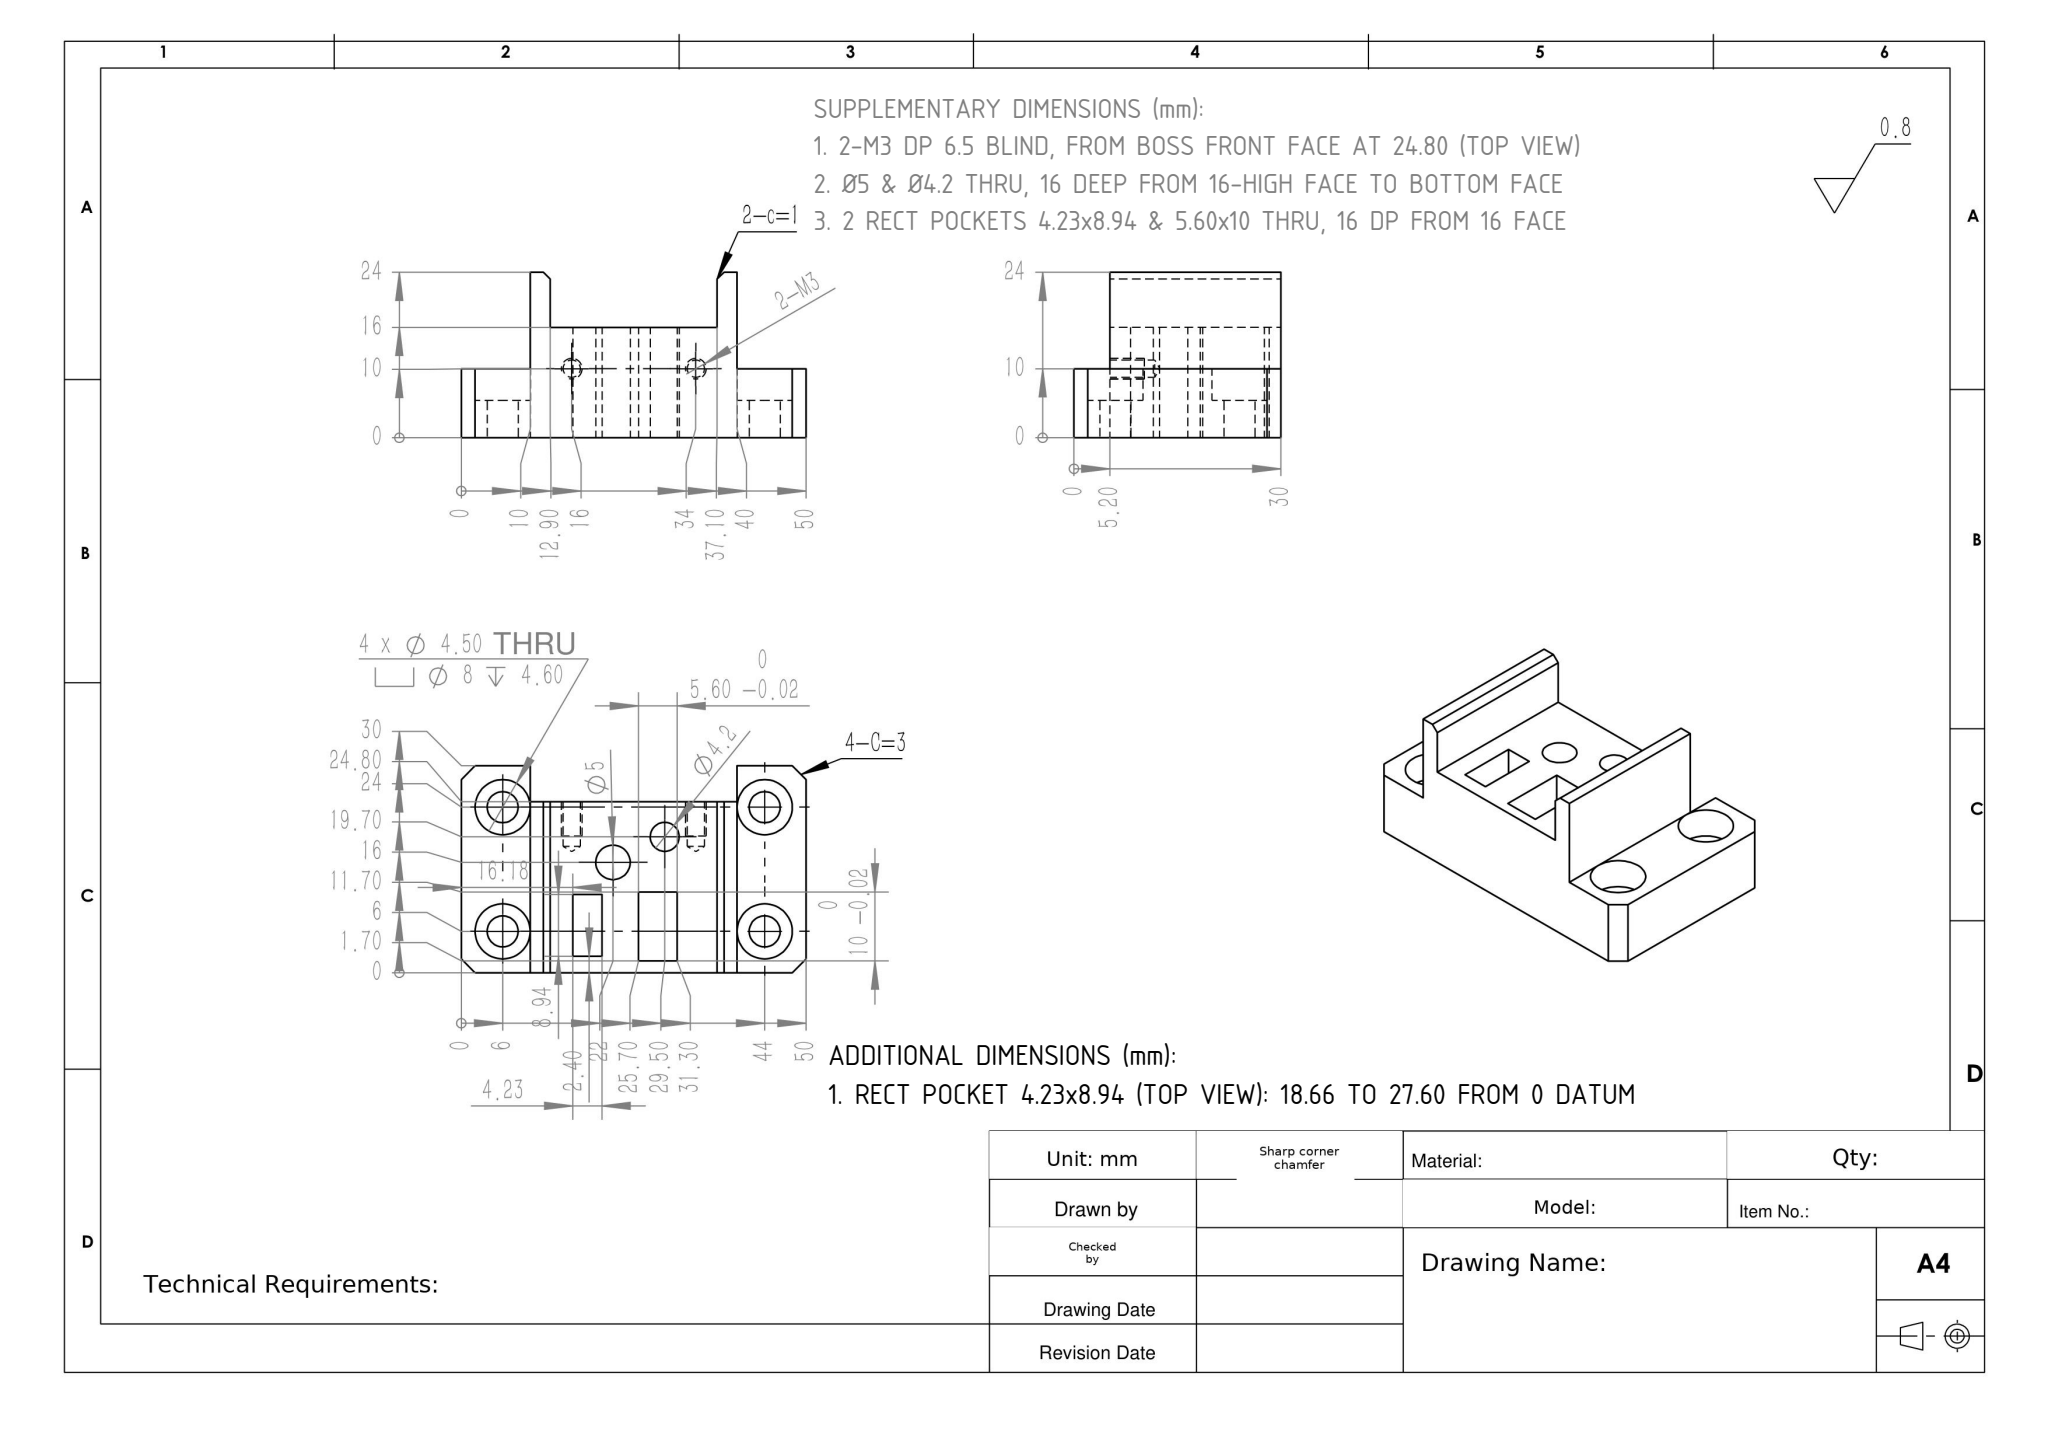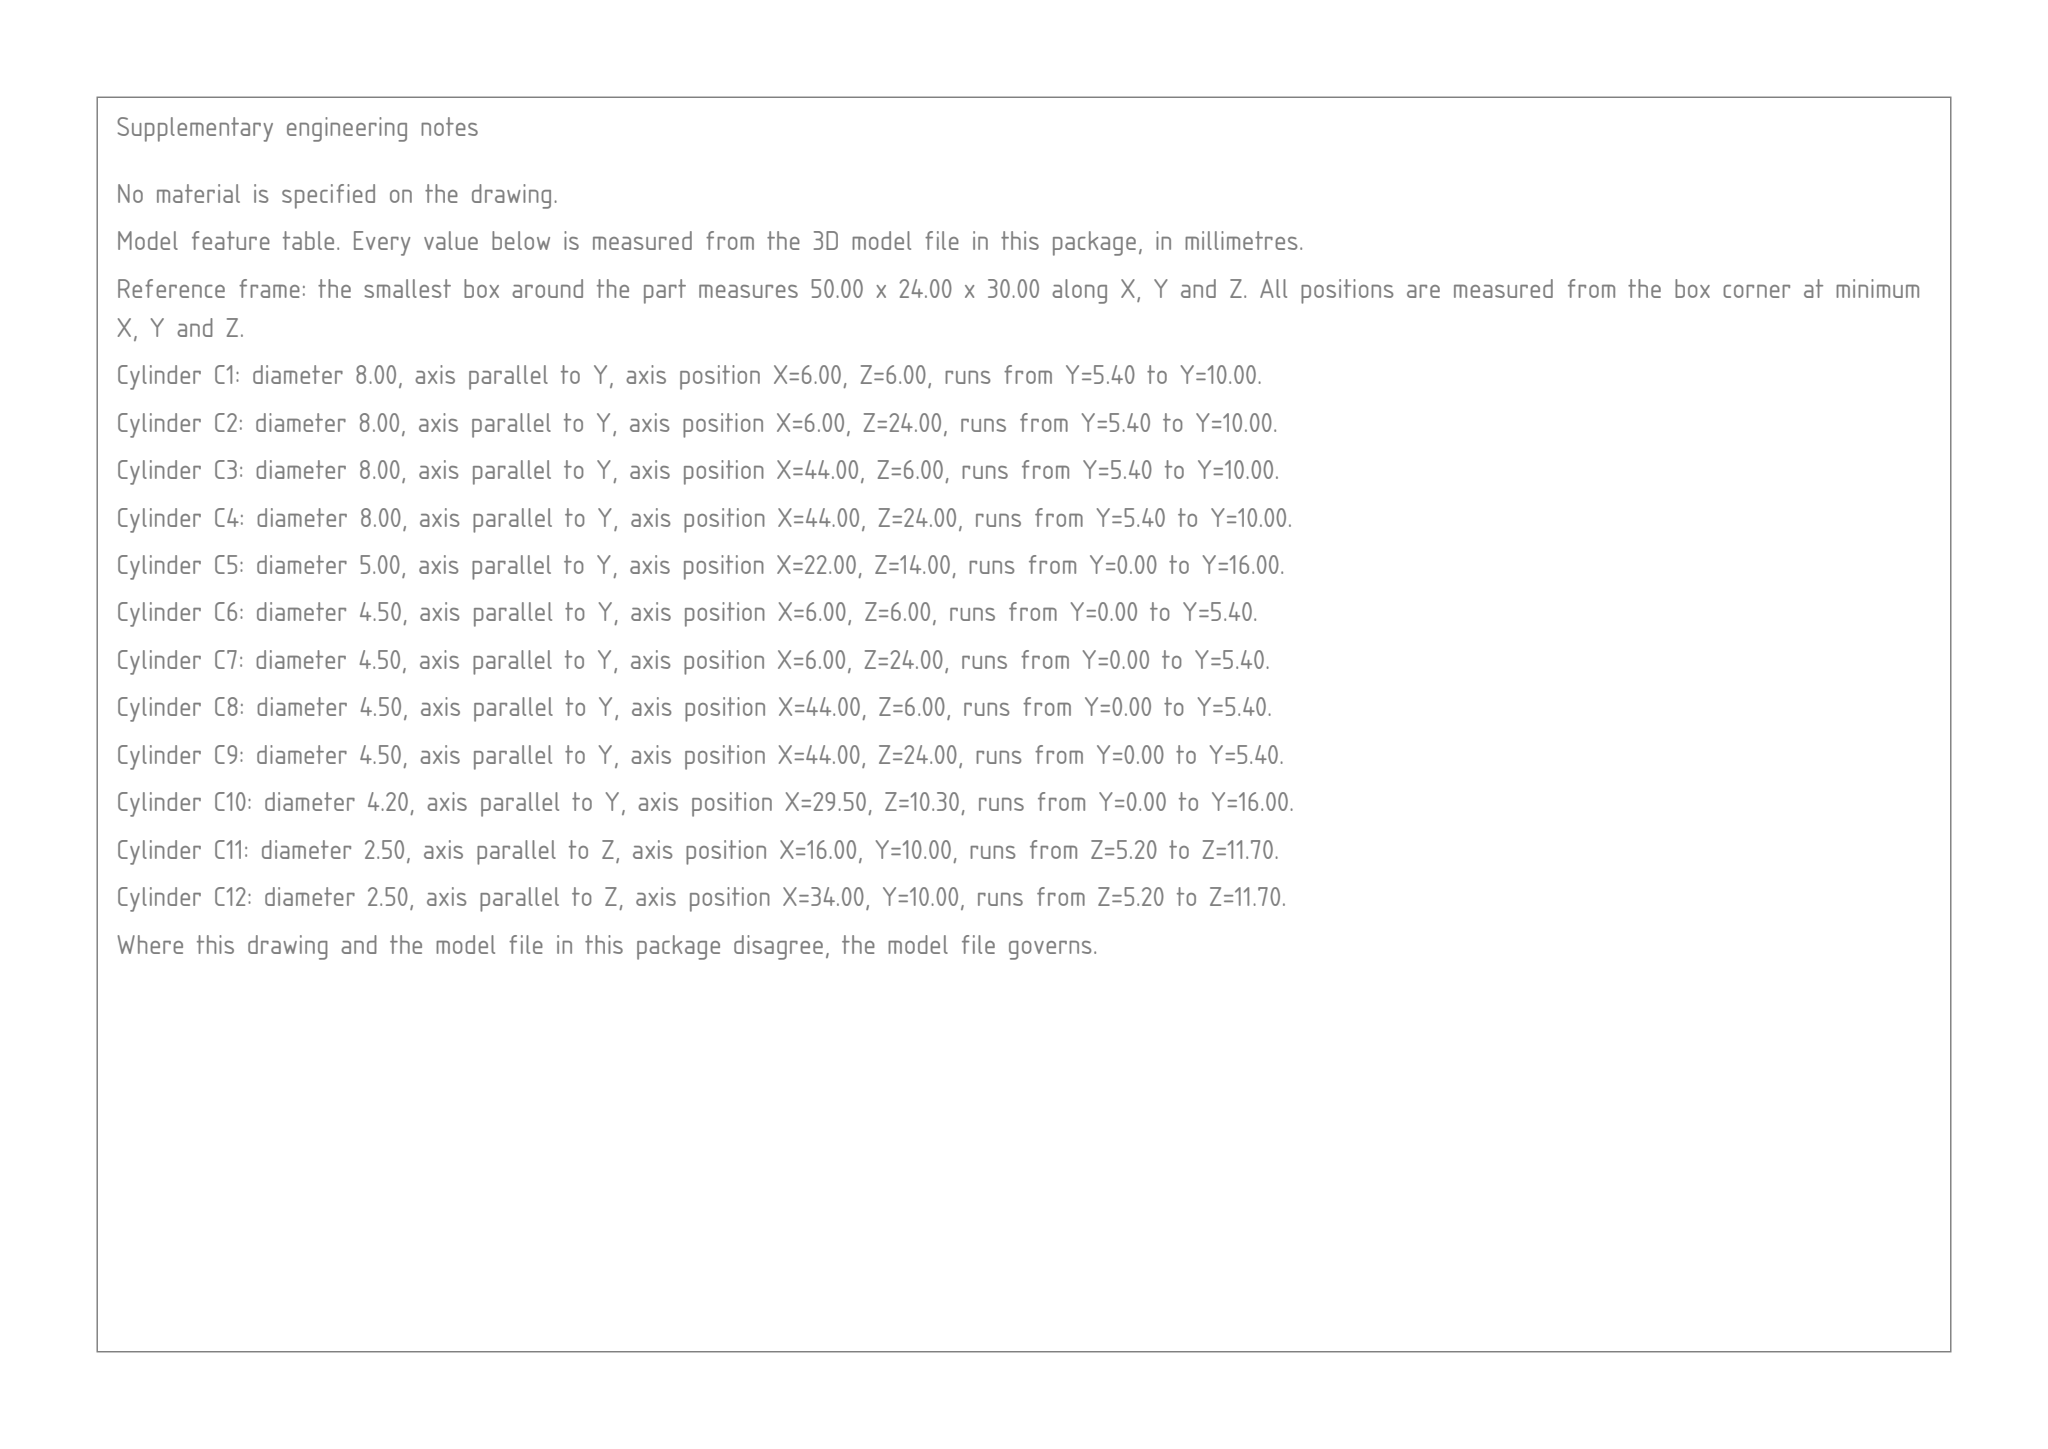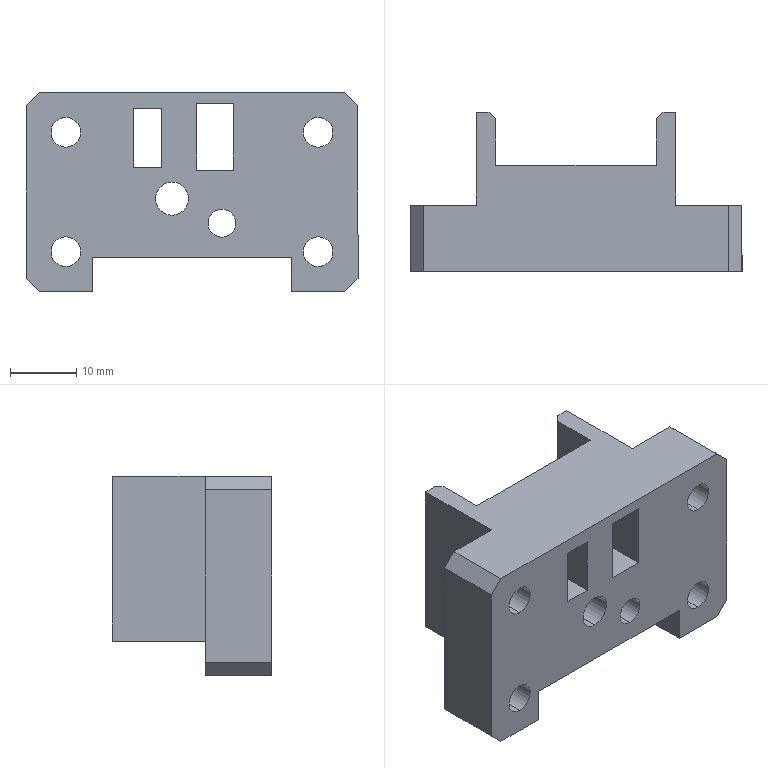Part | SolidWorks | mm | 1 solid | 64 faces | box 50 x 24 x 30 mm | volume 15578 mm3 | plane 36 | cylinder 24 | cone 4 | commonest cylinder face diameters 8 x8 4.5 x8 2.5 x4 5 x2 4.2 x2
build123d program:
from build123d import *

# Parameters (mm, degrees)
SKETCH1_W                                           = 50
SKETCH1_H                                           = 24
BOSS_EXTRUDE1_DEPTH                                 = 30
SKETCH2_W                                           = 10
SKETCH2_H                                           = 14
CUT_EXTRUDE1_DEPTH                                  = 64.056
SKETCH3_W                                           = 24.2
SKETCH3_H                                           = 8
CUT_EXTRUDE2_DEPTH                                  = 24.8
CHAMFER2_SIZE                                       = 2
SKETCH5_R                                           = 2.1
CUT_EXTRUDE3_DEPTH                                  = 64.056
HOLE_SIZE_TYPE_1_OF_SOCKET_HEAD_CAP_SCR_D           = 4.5
HOLE_SIZE_TYPE_1_OF_SOCKET_HEAD_CAP_SCR_CBORE_D     = 8
HOLE_SIZE_TYPE_1_OF_SOCKET_HEAD_CAP_SCR_CBORE_DEPTH = 4.6
CHAMFER3_SIZE                                       = 1
SKETCH12_W                                          = 5.6
SKETCH12_H                                          = 10
CUT_EXTRUDE5_DEPTH                                  = 61.465
SKETCH13_W                                          = 30
SKETCH13_H                                          = 5.2
CUT_EXTRUDE6_DEPTH                                  = 64.056
M3_TAPPED_HOLE1_D                                   = 2.5
M3_TAPPED_HOLE1_DEPTH                               = 6.5
M3_TAPPED_HOLE1_TIP                                 = 0.7511
CUT_EXTRUDE7_DEPTH                                  = 10
CUT_EXTRUDE7_DEPTH_BACK                             = 60.967
SKETCH16_R                                          = 2.5
SKETCH17_W                                          = 4.233
SKETCH17_H                                          = 8.941
CUT_EXTRUDE8_DEPTH                                  = 27


with BuildPart() as part:
    # Sketch1 → Boss-Extrude1 (new body)
    with BuildSketch(Plane.XY):
        with Locations((25, 12)):
            Rectangle(SKETCH1_W, SKETCH1_H)
    extrude(amount=BOSS_EXTRUDE1_DEPTH)

    # Sketch2 → Cut-Extrude1 (cut, through all)
    with BuildSketch(Plane.XY.offset(30)):
        with Locations((5, 17)):
            Rectangle(SKETCH2_W, SKETCH2_H)
        with Locations((45, 17)):
            Rectangle(SKETCH2_W, SKETCH2_H)
    extrude(amount=-CUT_EXTRUDE1_DEPTH, mode=Mode.SUBTRACT)

    # Sketch3 → Cut-Extrude2 (cut)
    with BuildSketch(Plane.XY.offset(30)):
        with Locations((25, 20)):
            Rectangle(SKETCH3_W, SKETCH3_H)
    extrude(amount=-CUT_EXTRUDE2_DEPTH, mode=Mode.SUBTRACT)

    # Chamfer2
    chamfer2_edges = [part.edges().sort_by_distance(p)[0] for p in [
        (50, 5, 30),
        (0, 5, 0),
        (0, 5, 30),
        (50, 5, 0),
    ]]
    chamfer(chamfer2_edges, length=CHAMFER2_SIZE)

    # Sketch5 → Cut-Extrude3 (cut, through all)
    with BuildSketch(Plane(origin=(0, 0, 0), x_dir=(-1, 0, 0), z_dir=(0, -1, 0))):
        with Locations(Location((-29.5, -10.3, 0), (0, 0, 90))):
            Circle(SKETCH5_R)
    extrude(amount=-CUT_EXTRUDE3_DEPTH, mode=Mode.SUBTRACT)

    # Hole Size _Type 1 of Socket Head Cap Scr (through all)
    with Locations(Plane(origin=(6, 10, 6), x_dir=(0, 0, 1), z_dir=(0, 1, 0))):
        with Locations((0, 0), (18, 0), (0, 38), (18, 38)):
            CounterBoreHole(HOLE_SIZE_TYPE_1_OF_SOCKET_HEAD_CAP_SCR_D / 2, HOLE_SIZE_TYPE_1_OF_SOCKET_HEAD_CAP_SCR_CBORE_D / 2, HOLE_SIZE_TYPE_1_OF_SOCKET_HEAD_CAP_SCR_CBORE_DEPTH)

    # Chamfer3
    chamfer3_edges = [part.edges().sort_by_distance(p)[0] for p in [
        (12.9, 24, 17.6),
        (37.1, 24, 17.6),
        (25, 24, 5.2),
    ]]
    chamfer(chamfer3_edges, length=CHAMFER3_SIZE)

    # Sketch12 → Cut-Extrude5 (cut, through all)
    with BuildSketch(Plane(origin=(0, 16, 0), x_dir=(1, 0, 0), z_dir=(0, 1, 0))):
        with Locations((28.5, -23.3)):
            Rectangle(SKETCH12_W, SKETCH12_H)
    extrude(amount=-CUT_EXTRUDE5_DEPTH, mode=Mode.SUBTRACT)

    # Sketch13 → Cut-Extrude6 (cut, through all)
    with BuildSketch(Plane(origin=(0, 24, 0), x_dir=(1, 0, 0), z_dir=(0, 1, 0))):
        with Locations((25, -2.6)):
            Rectangle(SKETCH13_W, SKETCH13_H)
    extrude(amount=-CUT_EXTRUDE6_DEPTH, mode=Mode.SUBTRACT)

    # M3 Tapped Hole1
    with Locations(Plane(origin=(34, 10, 5.2), x_dir=(-1, 0, 0), z_dir=(0, 0, -1))):
        with Locations((0, 0), (18, 0)):
            Hole(M3_TAPPED_HOLE1_D / 2, depth=M3_TAPPED_HOLE1_DEPTH)
            with Locations((0, 0, -(M3_TAPPED_HOLE1_DEPTH + M3_TAPPED_HOLE1_TIP / 2))):  # 118° drill point
                Cone(0, M3_TAPPED_HOLE1_D / 2, M3_TAPPED_HOLE1_TIP, mode=Mode.SUBTRACT)

    # Sketch16 → Cut-Extrude7 (cut, two sides: drawn at the far end of the back side and taken through both)
    with BuildSketch(Plane(origin=(0, 10, 0), x_dir=(1, 0, 0), z_dir=(0, 1, 0)).offset(-CUT_EXTRUDE7_DEPTH_BACK)):
        with Locations(Location((22, -14, 0), (0, 0, 90))):
            Circle(SKETCH16_R)
    extrude(amount=CUT_EXTRUDE7_DEPTH + CUT_EXTRUDE7_DEPTH_BACK, mode=Mode.SUBTRACT)

    # Sketch17 → Cut-Extrude8 (cut)
    with BuildSketch(Plane(origin=(0, 16, 0), x_dir=(1, 0, 0), z_dir=(0, 1, 0))):
        with Locations((18.294, -23.13)):
            Rectangle(SKETCH17_W, SKETCH17_H)
    extrude(amount=-CUT_EXTRUDE8_DEPTH, mode=Mode.SUBTRACT)


solid = part.part